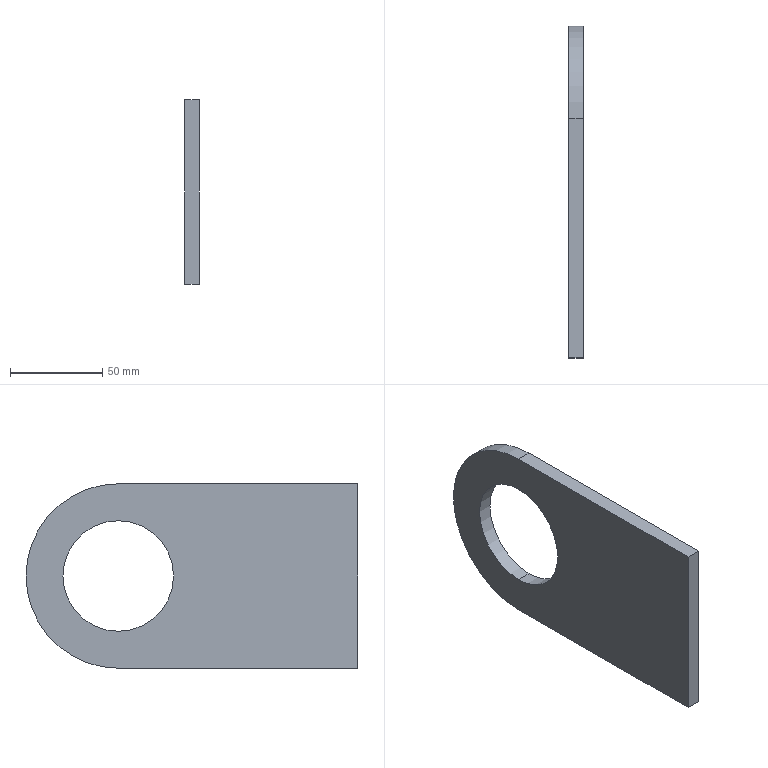Component | SolidWorks | 009LiftingLug-1 | 1 solid | 8 faces | box 8 x 180 x 100 mm | volume 112796 mm3 | plane 5 | cylinder 3 | commonest cylinder face diameters 60 x2 100 x1 | material Plain Carbon Steel
build123d program:
from build123d import *

# Parameters (mm, degrees)
SKETCH1_R           = 30
BOSS_EXTRUDE1_DEPTH = 4


with BuildPart() as part:
    # Sketch1 → Boss-Extrude1 (new, symmetric)
    with BuildSketch(Plane.XY):
        with BuildLine():
            Line((-50, 0), (-50, -130))
            Line((-50, -130), (50, -130))
            Line((50, -130), (50, 0))
            ThreePointArc((50, 0), (0, 50), (-50, 0))
        make_face()
        Circle(SKETCH1_R, mode=Mode.SUBTRACT)
    extrude(amount=BOSS_EXTRUDE1_DEPTH, both=True)


solid = part.part

# Placed as in the assembly
solid = solid.moved(Location((-49, 1437, -130), (0, 90, 0)))
STEP:
#1=COLOUR_RGB('',0.7922,0.8196,0.9333);
#2=FILL_AREA_STYLE_COLOUR('',#1);
#3=FILL_AREA_STYLE('',(#2));
#4=SURFACE_STYLE_FILL_AREA(#3);
#5=SURFACE_SIDE_STYLE('',(#4));
#6=SURFACE_STYLE_USAGE(.BOTH.,#5);
#7=PRESENTATION_STYLE_ASSIGNMENT((#6));
#8=CARTESIAN_POINT('',(-1.772,56.575,-3.937));
#9=VERTEX_POINT('',#8);
#10=CARTESIAN_POINT('',(-1.772,56.575,-6.299));
#11=VERTEX_POINT('',#10);
#12=CARTESIAN_POINT('',(-1.772,56.575,-5.118));
#13=DIRECTION('',(1.,0.,0.));
#14=DIRECTION('',(0.,0.,-1.));
#15=AXIS2_PLACEMENT_3D('',#12,#13,#14);
#16=CIRCLE('',#15,1.181);
#17=EDGE_CURVE('',#9,#11,#16,.T.);
#18=ORIENTED_EDGE('',*,*,#17,.T.);
#19=CARTESIAN_POINT('',(-2.087,56.575,-6.299));
#20=VERTEX_POINT('',#19);
#21=CARTESIAN_POINT('',(-1.772,56.575,-6.299));
#22=DIRECTION('',(-1.,0.,0.));
#23=VECTOR('',#22,39.37);
#24=LINE('',#21,#23);
#25=EDGE_CURVE('',#11,#20,#24,.T.);
#26=ORIENTED_EDGE('',*,*,#25,.T.);
#27=CARTESIAN_POINT('',(-2.087,56.575,-3.937));
#28=VERTEX_POINT('',#27);
#29=CARTESIAN_POINT('',(-2.087,56.575,-5.118));
#30=DIRECTION('',(1.,0.,0.));
#31=DIRECTION('',(0.,0.,-1.));
#32=AXIS2_PLACEMENT_3D('',#29,#30,#31);
#33=CIRCLE('',#32,1.181);
#34=EDGE_CURVE('',#28,#20,#33,.T.);
#35=ORIENTED_EDGE('',*,*,#34,.F.);
#36=CARTESIAN_POINT('',(-1.772,56.575,-3.937));
#37=DIRECTION('',(-1.,0.,0.));
#38=VECTOR('',#37,39.37);
#39=LINE('',#36,#38);
#40=EDGE_CURVE('',#9,#28,#39,.T.);
#41=ORIENTED_EDGE('',*,*,#40,.F.);
#42=EDGE_LOOP('',(#18,#26,#35,#41));
#43=FACE_OUTER_BOUND('',#42,.T.);
#44=CARTESIAN_POINT('',(-1.772,56.575,-5.118));
#45=DIRECTION('',(-1.,0.,0.));
#46=DIRECTION('',(0.,0.,1.));
#47=AXIS2_PLACEMENT_3D('',#44,#45,#46);
#48=CYLINDRICAL_SURFACE('',#47,1.181);
#49=ADVANCED_FACE('',(#43),#48,.F.);
#50=CARTESIAN_POINT('',(-1.772,56.575,-7.087));
#51=VERTEX_POINT('',#50);
#52=CARTESIAN_POINT('',(-1.772,56.575,-3.15));
#53=VERTEX_POINT('',#52);
#54=CARTESIAN_POINT('',(-1.772,56.575,-5.118));
#55=DIRECTION('',(1.,0.,0.));
#56=DIRECTION('',(0.,0.,-1.));
#57=AXIS2_PLACEMENT_3D('',#54,#55,#56);
#58=CIRCLE('',#57,1.969);
#59=EDGE_CURVE('',#51,#53,#58,.T.);
#60=ORIENTED_EDGE('',*,*,#59,.T.);
#61=CARTESIAN_POINT('',(-1.772,51.457,-3.15));
#62=VERTEX_POINT('',#61);
#63=CARTESIAN_POINT('',(-1.772,56.575,-3.15));
#64=DIRECTION('',(0.,-1.,-0.));
#65=VECTOR('',#64,39.37);
#66=LINE('',#63,#65);
#67=EDGE_CURVE('',#53,#62,#66,.T.);
#68=ORIENTED_EDGE('',*,*,#67,.T.);
#69=CARTESIAN_POINT('',(-1.772,51.457,-7.087));
#70=VERTEX_POINT('',#69);
#71=CARTESIAN_POINT('',(-1.772,51.457,-3.15));
#72=DIRECTION('',(0.,0.,-1.));
#73=VECTOR('',#72,39.37);
#74=LINE('',#71,#73);
#75=EDGE_CURVE('',#62,#70,#74,.T.);
#76=ORIENTED_EDGE('',*,*,#75,.T.);
#77=CARTESIAN_POINT('',(-1.772,51.457,-7.087));
#78=DIRECTION('',(0.,1.,-0.));
#79=VECTOR('',#78,39.37);
#80=LINE('',#77,#79);
#81=EDGE_CURVE('',#70,#51,#80,.T.);
#82=ORIENTED_EDGE('',*,*,#81,.T.);
#83=EDGE_LOOP('',(#60,#68,#76,#82));
#84=FACE_OUTER_BOUND('',#83,.T.);
#85=ORIENTED_EDGE('',*,*,#17,.F.);
#86=CARTESIAN_POINT('',(-1.772,56.575,-5.118));
#87=DIRECTION('',(1.,0.,0.));
#88=DIRECTION('',(0.,0.,-1.));
#89=AXIS2_PLACEMENT_3D('',#86,#87,#88);
#90=CIRCLE('',#89,1.181);
#91=EDGE_CURVE('',#11,#9,#90,.T.);
#92=ORIENTED_EDGE('',*,*,#91,.F.);
#93=EDGE_LOOP('',(#85,#92));
#94=FACE_BOUND('',#93,.T.);
#95=CARTESIAN_POINT('',(-1.772,56.575,-5.118));
#96=DIRECTION('',(1.,0.,0.));
#97=DIRECTION('',(0.,0.,-1.));
#98=AXIS2_PLACEMENT_3D('',#95,#96,#97);
#99=PLANE('',#98);
#100=ADVANCED_FACE('',(#84,#94),#99,.T.);
#101=CARTESIAN_POINT('',(-2.087,56.575,-7.087));
#102=VERTEX_POINT('',#101);
#103=CARTESIAN_POINT('',(-2.087,56.575,-3.15));
#104=VERTEX_POINT('',#103);
#105=CARTESIAN_POINT('',(-2.087,56.575,-5.118));
#106=DIRECTION('',(1.,0.,0.));
#107=DIRECTION('',(0.,0.,-1.));
#108=AXIS2_PLACEMENT_3D('',#105,#106,#107);
#109=CIRCLE('',#108,1.969);
#110=EDGE_CURVE('',#102,#104,#109,.T.);
#111=ORIENTED_EDGE('',*,*,#110,.F.);
#112=CARTESIAN_POINT('',(-2.087,51.457,-7.087));
#113=VERTEX_POINT('',#112);
#114=CARTESIAN_POINT('',(-2.087,51.457,-7.087));
#115=DIRECTION('',(0.,1.,-0.));
#116=VECTOR('',#115,39.37);
#117=LINE('',#114,#116);
#118=EDGE_CURVE('',#113,#102,#117,.T.);
#119=ORIENTED_EDGE('',*,*,#118,.F.);
#120=CARTESIAN_POINT('',(-2.087,51.457,-3.15));
#121=VERTEX_POINT('',#120);
#122=CARTESIAN_POINT('',(-2.087,51.457,-3.15));
#123=DIRECTION('',(0.,0.,-1.));
#124=VECTOR('',#123,39.37);
#125=LINE('',#122,#124);
#126=EDGE_CURVE('',#121,#113,#125,.T.);
#127=ORIENTED_EDGE('',*,*,#126,.F.);
#128=CARTESIAN_POINT('',(-2.087,56.575,-3.15));
#129=DIRECTION('',(0.,-1.,-0.));
#130=VECTOR('',#129,39.37);
#131=LINE('',#128,#130);
#132=EDGE_CURVE('',#104,#121,#131,.T.);
#133=ORIENTED_EDGE('',*,*,#132,.F.);
#134=EDGE_LOOP('',(#111,#119,#127,#133));
#135=FACE_OUTER_BOUND('',#134,.T.);
#136=ORIENTED_EDGE('',*,*,#34,.T.);
#137=CARTESIAN_POINT('',(-2.087,56.575,-5.118));
#138=DIRECTION('',(1.,0.,0.));
#139=DIRECTION('',(0.,0.,-1.));
#140=AXIS2_PLACEMENT_3D('',#137,#138,#139);
#141=CIRCLE('',#140,1.181);
#142=EDGE_CURVE('',#20,#28,#141,.T.);
#143=ORIENTED_EDGE('',*,*,#142,.T.);
#144=EDGE_LOOP('',(#136,#143));
#145=FACE_BOUND('',#144,.T.);
#146=CARTESIAN_POINT('',(-2.087,56.575,-5.118));
#147=DIRECTION('',(1.,0.,0.));
#148=DIRECTION('',(0.,0.,-1.));
#149=AXIS2_PLACEMENT_3D('',#146,#147,#148);
#150=PLANE('',#149);
#151=ADVANCED_FACE('',(#135,#145),#150,.F.);
#152=ORIENTED_EDGE('',*,*,#110,.T.);
#153=CARTESIAN_POINT('',(-1.772,56.575,-3.15));
#154=DIRECTION('',(-1.,0.,0.));
#155=VECTOR('',#154,39.37);
#156=LINE('',#153,#155);
#157=EDGE_CURVE('',#53,#104,#156,.T.);
#158=ORIENTED_EDGE('',*,*,#157,.F.);
#159=ORIENTED_EDGE('',*,*,#59,.F.);
#160=CARTESIAN_POINT('',(-1.772,56.575,-7.087));
#161=DIRECTION('',(-1.,0.,0.));
#162=VECTOR('',#161,39.37);
#163=LINE('',#160,#162);
#164=EDGE_CURVE('',#51,#102,#163,.T.);
#165=ORIENTED_EDGE('',*,*,#164,.T.);
#166=EDGE_LOOP('',(#152,#158,#159,#165));
#167=FACE_OUTER_BOUND('',#166,.T.);
#168=CARTESIAN_POINT('',(-1.772,56.575,-5.118));
#169=DIRECTION('',(-1.,0.,0.));
#170=DIRECTION('',(0.,0.,1.));
#171=AXIS2_PLACEMENT_3D('',#168,#169,#170);
#172=CYLINDRICAL_SURFACE('',#171,1.969);
#173=ADVANCED_FACE('',(#167),#172,.T.);
#174=ORIENTED_EDGE('',*,*,#132,.T.);
#175=CARTESIAN_POINT('',(-1.772,51.457,-3.15));
#176=DIRECTION('',(-1.,0.,0.));
#177=VECTOR('',#176,39.37);
#178=LINE('',#175,#177);
#179=EDGE_CURVE('',#62,#121,#178,.T.);
#180=ORIENTED_EDGE('',*,*,#179,.F.);
#181=ORIENTED_EDGE('',*,*,#67,.F.);
#182=ORIENTED_EDGE('',*,*,#157,.T.);
#183=EDGE_LOOP('',(#174,#180,#181,#182));
#184=FACE_OUTER_BOUND('',#183,.T.);
#185=CARTESIAN_POINT('',(-1.772,56.575,-3.15));
#186=DIRECTION('',(0.,0.,-1.));
#187=DIRECTION('',(0.,1.,0.));
#188=AXIS2_PLACEMENT_3D('',#185,#186,#187);
#189=PLANE('',#188);
#190=ADVANCED_FACE('',(#184),#189,.F.);
#191=ORIENTED_EDGE('',*,*,#126,.T.);
#192=CARTESIAN_POINT('',(-1.772,51.457,-7.087));
#193=DIRECTION('',(-1.,0.,0.));
#194=VECTOR('',#193,39.37);
#195=LINE('',#192,#194);
#196=EDGE_CURVE('',#70,#113,#195,.T.);
#197=ORIENTED_EDGE('',*,*,#196,.F.);
#198=ORIENTED_EDGE('',*,*,#75,.F.);
#199=ORIENTED_EDGE('',*,*,#179,.T.);
#200=EDGE_LOOP('',(#191,#197,#198,#199));
#201=FACE_OUTER_BOUND('',#200,.T.);
#202=CARTESIAN_POINT('',(-1.772,51.457,-3.15));
#203=DIRECTION('',(0.,1.,0.));
#204=DIRECTION('',(1.,0.,0.));
#205=AXIS2_PLACEMENT_3D('',#202,#203,#204);
#206=PLANE('',#205);
#207=ADVANCED_FACE('',(#201),#206,.F.);
#208=ORIENTED_EDGE('',*,*,#118,.T.);
#209=ORIENTED_EDGE('',*,*,#164,.F.);
#210=ORIENTED_EDGE('',*,*,#81,.F.);
#211=ORIENTED_EDGE('',*,*,#196,.T.);
#212=EDGE_LOOP('',(#208,#209,#210,#211));
#213=FACE_OUTER_BOUND('',#212,.T.);
#214=CARTESIAN_POINT('',(-1.772,51.457,-7.087));
#215=DIRECTION('',(0.,0.,1.));
#216=DIRECTION('',(0.,-1.,0.));
#217=AXIS2_PLACEMENT_3D('',#214,#215,#216);
#218=PLANE('',#217);
#219=ADVANCED_FACE('',(#213),#218,.F.);
#220=ORIENTED_EDGE('',*,*,#25,.F.);
#221=ORIENTED_EDGE('',*,*,#91,.T.);
#222=ORIENTED_EDGE('',*,*,#40,.T.);
#223=ORIENTED_EDGE('',*,*,#142,.F.);
#224=EDGE_LOOP('',(#220,#221,#222,#223));
#225=FACE_OUTER_BOUND('',#224,.T.);
#226=CARTESIAN_POINT('',(-1.772,56.575,-5.118));
#227=DIRECTION('',(-1.,0.,0.));
#228=DIRECTION('',(0.,0.,1.));
#229=AXIS2_PLACEMENT_3D('',#226,#227,#228);
#230=CYLINDRICAL_SURFACE('',#229,1.181);
#231=ADVANCED_FACE('',(#225),#230,.F.);
#232=CLOSED_SHELL('',(#49,#100,#151,#173,#190,#207,#219,#231));
#233=MANIFOLD_SOLID_BREP('',#232);
#234=STYLED_ITEM('',(#7),#233);
#235=PRESENTATION_LAYER_ASSIGNMENT('','',(#234));
#236=(LENGTH_UNIT()NAMED_UNIT(*)SI_UNIT($,.METRE.));
#237=LENGTH_MEASURE_WITH_UNIT(LENGTH_MEASURE(0.0254),#236);
#238=DIMENSIONAL_EXPONENTS(1.,0.,0.,0.,0.,0.,0.);
#239=(CONVERSION_BASED_UNIT('',#237)LENGTH_UNIT()NAMED_UNIT(#238));
#240=UNCERTAINTY_MEASURE_WITH_UNIT(LENGTH_MEASURE(0.00001),#239,'','');
#241=(NAMED_UNIT(*)PLANE_ANGLE_UNIT()SI_UNIT($,.RADIAN.));
#242=(NAMED_UNIT(*)SI_UNIT($,.STERADIAN.)SOLID_ANGLE_UNIT());
#243=(GEOMETRIC_REPRESENTATION_CONTEXT(3)GLOBAL_UNCERTAINTY_ASSIGNED_CONTEXT((#240))GLOBAL_UNIT_ASSIGNED_CONTEXT((#239,#241,#242))REPRESENTATION_CONTEXT('',''));
#244=MECHANICAL_DESIGN_GEOMETRIC_PRESENTATION_REPRESENTATION('',(#234),#243);
#245=CARTESIAN_POINT('',(0.,0.,0.));
#246=DIRECTION('',(0.,0.,1.));
#247=DIRECTION('',(1.,0.,0.));
#248=AXIS2_PLACEMENT_3D('',#245,#246,#247);
#249=(LENGTH_UNIT()NAMED_UNIT(*)SI_UNIT($,.METRE.));
#250=LENGTH_MEASURE_WITH_UNIT(LENGTH_MEASURE(0.0254),#249);
#251=DIMENSIONAL_EXPONENTS(1.,0.,0.,0.,0.,0.,0.);
#252=(CONVERSION_BASED_UNIT('',#250)LENGTH_UNIT()NAMED_UNIT(#251));
#253=UNCERTAINTY_MEASURE_WITH_UNIT(LENGTH_MEASURE(0.00001),#252,'','');
#254=(NAMED_UNIT(*)PLANE_ANGLE_UNIT()SI_UNIT($,.RADIAN.));
#255=(NAMED_UNIT(*)SI_UNIT($,.STERADIAN.)SOLID_ANGLE_UNIT());
#256=(GEOMETRIC_REPRESENTATION_CONTEXT(3)GLOBAL_UNCERTAINTY_ASSIGNED_CONTEXT((#253))GLOBAL_UNIT_ASSIGNED_CONTEXT((#252,#254,#255))REPRESENTATION_CONTEXT('',''));
#257=ADVANCED_BREP_SHAPE_REPRESENTATION('',(#233,#248),#256);